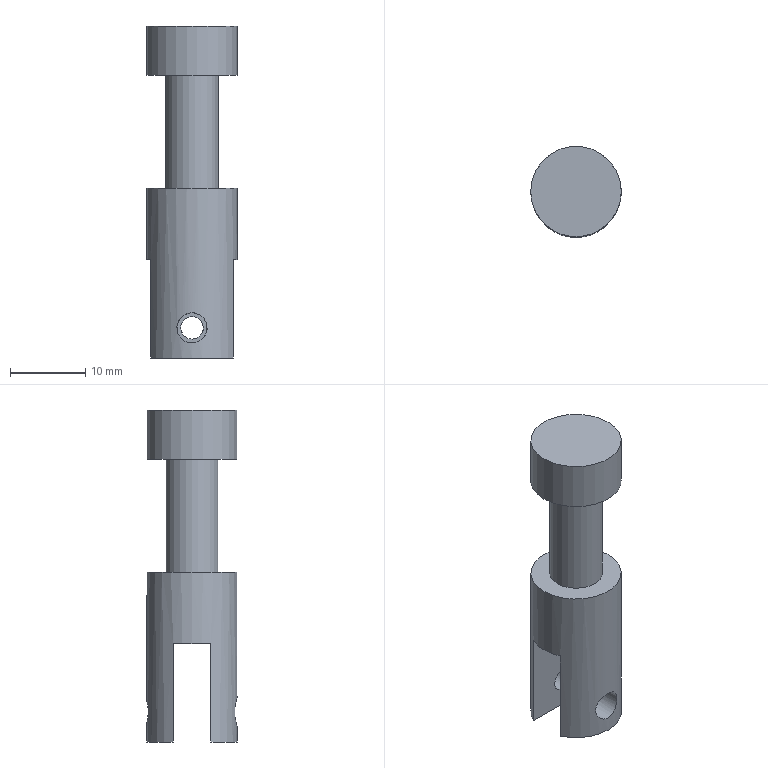Component | NX | SMALL_PISTON | 1 solid | 13 faces | volume 3033 mm3 | plane 8 | cylinder 5 | commonest cylinder face diameters 12 x2 7 x1 4 x1 3 x1